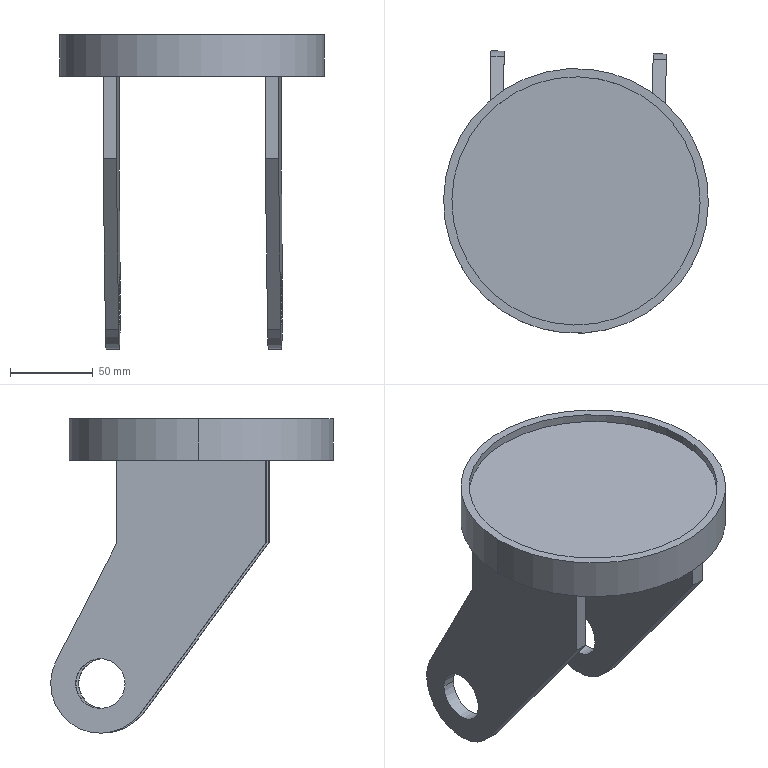Component | SolidWorks | FrontWheelAssembly-1_FrontWheelAccessory2-1 | 1 solid | 26 faces | box 160 x 170.95 x 190 mm | volume 607648 mm3 | plane 15 | cylinder 11 | commonest cylinder face diameters 30 x4 60 x3 150 x2 160 x2
build123d program:
from build123d import *

# Parameters (mm, degrees)
SKETCH1_R           = 80
SKETCH1_R_2         = 75
BOSS_EXTRUDE1_DEPTH = 5
BOSS_EXTRUDE2_START = 20
SKETCH2_R           = 80
BOSS_EXTRUDE2_DEPTH = 20
SKETCH3_R           = 15
BOSS_EXTRUDE3_DEPTH = 8


with BuildPart() as part:
    # Sketch1 → Boss-Extrude1 (new body)
    with BuildSketch(Plane(origin=(0, 0, 0), x_dir=(1, 0, 0), z_dir=(0, 1, 0))):
        with Locations(Location((0, 0, 0), (0, 0, 270))):
            Circle(SKETCH1_R)
        with Locations(Location((0, 0, 0), (0, 0, 270))):
            Circle(SKETCH1_R_2, mode=Mode.SUBTRACT)
    extrude(amount=BOSS_EXTRUDE1_DEPTH)

    # Sketch2 → Boss-Extrude2 (add)
    with BuildSketch(Plane.XZ.offset(BOSS_EXTRUDE2_START)):
        with Locations(Location((0, 0, 0), (0, 0, 270))):
            Circle(SKETCH2_R)
    extrude(amount=-BOSS_EXTRUDE2_DEPTH)

    # Sketch3 → Boss-Extrude3 (add)
    with BuildSketch(Plane.XY.offset(45)):
        with BuildLine():
            Line((50, -70), (50, -20))
            Line((50, -20), (-40.058, -20))
            Line((-40.058, -20), (-40.058, -70))
            Line((-40.058, -70), (35.866, -172.821))
            ThreePointArc((35.866, -172.821), (75.825, -180.487), (86.676, -141.273))
            Line((86.676, -141.273), (50, -70))
        make_face()
        with Locations((60, -155)):
            Circle(SKETCH3_R, mode=Mode.SUBTRACT)
    boss_extrude3 = extrude(amount=BOSS_EXTRUDE3_DEPTH)

    # Mirror1: Boss-Extrude3 across plane
    add(boss_extrude3.mirror(Plane.XY))


solid = part.part

# Placed as in the assembly
solid = solid.moved(Location((25.629, -64.9, 223), (90, 88.961, 0)))
STEP:
#1=COLOUR_RGB('',0.7922,0.8196,0.9333);
#2=FILL_AREA_STYLE_COLOUR('',#1);
#3=FILL_AREA_STYLE('',(#2));
#4=SURFACE_STYLE_FILL_AREA(#3);
#5=SURFACE_SIDE_STYLE('',(#4));
#6=SURFACE_STYLE_USAGE(.BOTH.,#5);
#7=PRESENTATION_STYLE_ASSIGNMENT((#6));
#8=CARTESIAN_POINT('',(-1.045,-0.7459,2.677));
#9=VERTEX_POINT('',#8);
#10=CARTESIAN_POINT('',(-1.024,0.435,2.677));
#11=VERTEX_POINT('',#10);
#12=CARTESIAN_POINT('',(-1.034,-0.1555,2.677));
#13=DIRECTION('',(0.9998,-0.01813,0.));
#14=DIRECTION('',(0.01813,0.9998,0.));
#15=AXIS2_PLACEMENT_3D('',#12,#13,#14);
#16=CIRCLE('',#15,0.5906);
#17=EDGE_CURVE('',#9,#11,#16,.T.);
#18=ORIENTED_EDGE('',*,*,#17,.F.);
#19=CARTESIAN_POINT('',(-0.7302,-0.7516,2.677));
#20=VERTEX_POINT('',#19);
#21=CARTESIAN_POINT('',(-1.045,-0.7459,2.677));
#22=DIRECTION('',(0.9998,-0.01813,0.));
#23=VECTOR('',#22,39.37);
#24=LINE('',#21,#23);
#25=EDGE_CURVE('',#9,#20,#24,.T.);
#26=ORIENTED_EDGE('',*,*,#25,.T.);
#27=CARTESIAN_POINT('',(-0.7088,0.4293,2.677));
#28=VERTEX_POINT('',#27);
#29=CARTESIAN_POINT('',(-0.7195,-0.1612,2.677));
#30=DIRECTION('',(0.9998,-0.01813,0.));
#31=DIRECTION('',(0.01813,0.9998,0.));
#32=AXIS2_PLACEMENT_3D('',#29,#30,#31);
#33=CIRCLE('',#32,0.5906);
#34=EDGE_CURVE('',#20,#28,#33,.T.);
#35=ORIENTED_EDGE('',*,*,#34,.T.);
#36=CARTESIAN_POINT('',(-1.024,0.435,2.677));
#37=DIRECTION('',(0.9998,-0.01813,0.));
#38=VECTOR('',#37,39.37);
#39=LINE('',#36,#38);
#40=EDGE_CURVE('',#11,#28,#39,.T.);
#41=ORIENTED_EDGE('',*,*,#40,.F.);
#42=EDGE_LOOP('',(#18,#26,#35,#41));
#43=FACE_OUTER_BOUND('',#42,.T.);
#44=CARTESIAN_POINT('',(-1.034,-0.1555,2.677));
#45=DIRECTION('',(0.9998,-0.01813,0.));
#46=DIRECTION('',(0.01813,0.9998,0.));
#47=AXIS2_PLACEMENT_3D('',#44,#45,#46);
#48=CYLINDRICAL_SURFACE('',#47,0.5906);
#49=ADVANCED_FACE('',(#43),#48,.F.);
#50=CARTESIAN_POINT('',(-1.052,-1.105,1.976));
#51=VERTEX_POINT('',#50);
#52=CARTESIAN_POINT('',(-1.013,1.025,2.677));
#53=VERTEX_POINT('',#52);
#54=CARTESIAN_POINT('',(-1.034,-0.1555,2.677));
#55=DIRECTION('',(0.9998,-0.01813,0.));
#56=DIRECTION('',(0.01813,0.9998,0.));
#57=AXIS2_PLACEMENT_3D('',#54,#55,#56);
#58=CIRCLE('',#57,1.181);
#59=EDGE_CURVE('',#51,#53,#58,.T.);
#60=ORIENTED_EDGE('',*,*,#59,.T.);
#61=CARTESIAN_POINT('',(-0.6981,1.02,2.677));
#62=VERTEX_POINT('',#61);
#63=CARTESIAN_POINT('',(-1.013,1.025,2.677));
#64=DIRECTION('',(0.9998,-0.01813,0.));
#65=VECTOR('',#64,39.37);
#66=LINE('',#63,#65);
#67=EDGE_CURVE('',#53,#62,#66,.T.);
#68=ORIENTED_EDGE('',*,*,#67,.T.);
#69=CARTESIAN_POINT('',(-0.7367,-1.111,1.976));
#70=VERTEX_POINT('',#69);
#71=CARTESIAN_POINT('',(-0.7195,-0.1612,2.677));
#72=DIRECTION('',(0.9998,-0.01813,0.));
#73=DIRECTION('',(0.01813,0.9998,0.));
#74=AXIS2_PLACEMENT_3D('',#71,#72,#73);
#75=CIRCLE('',#74,1.181);
#76=EDGE_CURVE('',#70,#62,#75,.T.);
#77=ORIENTED_EDGE('',*,*,#76,.F.);
#78=CARTESIAN_POINT('',(-1.052,-1.105,1.976));
#79=DIRECTION('',(0.9998,-0.01813,0.));
#80=VECTOR('',#79,39.37);
#81=LINE('',#78,#80);
#82=EDGE_CURVE('',#51,#70,#81,.T.);
#83=ORIENTED_EDGE('',*,*,#82,.F.);
#84=EDGE_LOOP('',(#60,#68,#77,#83));
#85=FACE_OUTER_BOUND('',#84,.T.);
#86=CARTESIAN_POINT('',(-1.034,-0.1555,2.677));
#87=DIRECTION('',(0.9998,-0.01813,0.));
#88=DIRECTION('',(0.01813,0.9998,0.));
#89=AXIS2_PLACEMENT_3D('',#86,#87,#88);
#90=CYLINDRICAL_SURFACE('',#89,1.181);
#91=ADVANCED_FACE('',(#85),#90,.T.);
#92=CARTESIAN_POINT('',(3.127,-0.8216,2.677));
#93=VERTEX_POINT('',#92);
#94=CARTESIAN_POINT('',(3.149,0.3593,2.677));
#95=VERTEX_POINT('',#94);
#96=CARTESIAN_POINT('',(3.138,-0.2311,2.677));
#97=DIRECTION('',(0.9998,-0.01813,0.));
#98=DIRECTION('',(0.01813,0.9998,0.));
#99=AXIS2_PLACEMENT_3D('',#96,#97,#98);
#100=CIRCLE('',#99,0.5906);
#101=EDGE_CURVE('',#93,#95,#100,.T.);
#102=ORIENTED_EDGE('',*,*,#101,.T.);
#103=CARTESIAN_POINT('',(2.834,0.365,2.677));
#104=VERTEX_POINT('',#103);
#105=CARTESIAN_POINT('',(3.149,0.3593,2.677));
#106=DIRECTION('',(-0.9998,0.01813,-0.));
#107=VECTOR('',#106,39.37);
#108=LINE('',#105,#107);
#109=EDGE_CURVE('',#95,#104,#108,.T.);
#110=ORIENTED_EDGE('',*,*,#109,.T.);
#111=CARTESIAN_POINT('',(2.813,-0.8159,2.677));
#112=VERTEX_POINT('',#111);
#113=CARTESIAN_POINT('',(2.823,-0.2254,2.677));
#114=DIRECTION('',(0.9998,-0.01813,0.));
#115=DIRECTION('',(0.01813,0.9998,0.));
#116=AXIS2_PLACEMENT_3D('',#113,#114,#115);
#117=CIRCLE('',#116,0.5906);
#118=EDGE_CURVE('',#112,#104,#117,.T.);
#119=ORIENTED_EDGE('',*,*,#118,.F.);
#120=CARTESIAN_POINT('',(3.127,-0.8216,2.677));
#121=DIRECTION('',(-0.9998,0.01813,-0.));
#122=VECTOR('',#121,39.37);
#123=LINE('',#120,#122);
#124=EDGE_CURVE('',#93,#112,#123,.T.);
#125=ORIENTED_EDGE('',*,*,#124,.F.);
#126=EDGE_LOOP('',(#102,#110,#119,#125));
#127=FACE_OUTER_BOUND('',#126,.T.);
#128=CARTESIAN_POINT('',(3.138,-0.2311,2.677));
#129=DIRECTION('',(-0.9998,0.01813,-0.));
#130=DIRECTION('',(-0.01813,-0.9998,-0.));
#131=AXIS2_PLACEMENT_3D('',#128,#129,#130);
#132=CYLINDRICAL_SURFACE('',#131,0.5906);
#133=ADVANCED_FACE('',(#127),#132,.F.);
#134=CARTESIAN_POINT('',(-1.943,-2.502,8.976));
#135=VERTEX_POINT('',#134);
#136=CARTESIAN_POINT('',(3.961,-2.609,8.976));
#137=VERTEX_POINT('',#136);
#138=CARTESIAN_POINT('',(1.009,-2.555,8.976));
#139=DIRECTION('',(-0.,-0.,1.));
#140=DIRECTION('',(0.9998,-0.01813,0.));
#141=AXIS2_PLACEMENT_3D('',#138,#139,#140);
#142=CIRCLE('',#141,2.953);
#143=EDGE_CURVE('',#135,#137,#142,.T.);
#144=ORIENTED_EDGE('',*,*,#143,.T.);
#145=CARTESIAN_POINT('',(3.961,-2.609,8.78));
#146=VERTEX_POINT('',#145);
#147=CARTESIAN_POINT('',(3.961,-2.609,8.976));
#148=DIRECTION('',(0.,0.,-1.));
#149=VECTOR('',#148,39.37);
#150=LINE('',#147,#149);
#151=EDGE_CURVE('',#137,#146,#150,.T.);
#152=ORIENTED_EDGE('',*,*,#151,.T.);
#153=CARTESIAN_POINT('',(-1.943,-2.502,8.78));
#154=VERTEX_POINT('',#153);
#155=CARTESIAN_POINT('',(1.009,-2.555,8.78));
#156=DIRECTION('',(-0.,-0.,1.));
#157=DIRECTION('',(0.9998,-0.01813,0.));
#158=AXIS2_PLACEMENT_3D('',#155,#156,#157);
#159=CIRCLE('',#158,2.953);
#160=EDGE_CURVE('',#154,#146,#159,.T.);
#161=ORIENTED_EDGE('',*,*,#160,.F.);
#162=CARTESIAN_POINT('',(-1.943,-2.502,8.976));
#163=DIRECTION('',(0.,0.,-1.));
#164=VECTOR('',#163,39.37);
#165=LINE('',#162,#164);
#166=EDGE_CURVE('',#135,#154,#165,.T.);
#167=ORIENTED_EDGE('',*,*,#166,.F.);
#168=EDGE_LOOP('',(#144,#152,#161,#167));
#169=FACE_OUTER_BOUND('',#168,.T.);
#170=CARTESIAN_POINT('',(1.009,-2.555,8.976));
#171=DIRECTION('',(0.,0.,-1.));
#172=DIRECTION('',(-0.9998,0.01813,-0.));
#173=AXIS2_PLACEMENT_3D('',#170,#171,#172);
#174=CYLINDRICAL_SURFACE('',#173,2.953);
#175=ADVANCED_FACE('',(#169),#174,.F.);
#176=CARTESIAN_POINT('',(4.158,-2.612,8.976));
#177=VERTEX_POINT('',#176);
#178=CARTESIAN_POINT('',(-2.14,-2.498,8.976));
#179=VERTEX_POINT('',#178);
#180=CARTESIAN_POINT('',(1.009,-2.555,8.976));
#181=DIRECTION('',(-0.,-0.,1.));
#182=DIRECTION('',(0.9998,-0.01813,0.));
#183=AXIS2_PLACEMENT_3D('',#180,#181,#182);
#184=CIRCLE('',#183,3.15);
#185=EDGE_CURVE('',#177,#179,#184,.T.);
#186=ORIENTED_EDGE('',*,*,#185,.F.);
#187=CARTESIAN_POINT('',(4.158,-2.612,7.992));
#188=VERTEX_POINT('',#187);
#189=CARTESIAN_POINT('',(4.158,-2.612,8.976));
#190=DIRECTION('',(0.,0.,-1.));
#191=VECTOR('',#190,39.37);
#192=LINE('',#189,#191);
#193=EDGE_CURVE('',#177,#188,#192,.T.);
#194=ORIENTED_EDGE('',*,*,#193,.T.);
#195=CARTESIAN_POINT('',(-2.14,-2.498,7.992));
#196=VERTEX_POINT('',#195);
#197=CARTESIAN_POINT('',(1.009,-2.555,7.992));
#198=DIRECTION('',(0.,0.,-1.));
#199=DIRECTION('',(-0.9998,0.01813,-0.));
#200=AXIS2_PLACEMENT_3D('',#197,#198,#199);
#201=CIRCLE('',#200,3.15);
#202=EDGE_CURVE('',#196,#188,#201,.T.);
#203=ORIENTED_EDGE('',*,*,#202,.F.);
#204=CARTESIAN_POINT('',(-2.14,-2.498,8.976));
#205=DIRECTION('',(0.,0.,-1.));
#206=VECTOR('',#205,39.37);
#207=LINE('',#204,#206);
#208=EDGE_CURVE('',#179,#196,#207,.T.);
#209=ORIENTED_EDGE('',*,*,#208,.F.);
#210=EDGE_LOOP('',(#186,#194,#203,#209));
#211=FACE_OUTER_BOUND('',#210,.T.);
#212=CARTESIAN_POINT('',(1.009,-2.555,8.976));
#213=DIRECTION('',(0.,0.,-1.));
#214=DIRECTION('',(-0.9998,0.01813,-0.));
#215=AXIS2_PLACEMENT_3D('',#212,#213,#214);
#216=CYLINDRICAL_SURFACE('',#215,3.15);
#217=ADVANCED_FACE('',(#211),#216,.T.);
#218=CARTESIAN_POINT('',(1.009,-2.555,8.976));
#219=DIRECTION('',(-0.,-0.,1.));
#220=DIRECTION('',(0.9998,-0.01813,0.));
#221=AXIS2_PLACEMENT_3D('',#218,#219,#220);
#222=CIRCLE('',#221,3.15);
#223=EDGE_CURVE('',#179,#177,#222,.T.);
#224=ORIENTED_EDGE('',*,*,#223,.T.);
#225=ORIENTED_EDGE('',*,*,#185,.T.);
#226=EDGE_LOOP('',(#224,#225));
#227=FACE_OUTER_BOUND('',#226,.T.);
#228=ORIENTED_EDGE('',*,*,#143,.F.);
#229=CARTESIAN_POINT('',(1.009,-2.555,8.976));
#230=DIRECTION('',(-0.,-0.,1.));
#231=DIRECTION('',(0.9998,-0.01813,0.));
#232=AXIS2_PLACEMENT_3D('',#229,#230,#231);
#233=CIRCLE('',#232,2.953);
#234=EDGE_CURVE('',#137,#135,#233,.T.);
#235=ORIENTED_EDGE('',*,*,#234,.F.);
#236=EDGE_LOOP('',(#228,#235));
#237=FACE_BOUND('',#236,.T.);
#238=CARTESIAN_POINT('',(1.009,-2.555,8.976));
#239=DIRECTION('',(-0.,-0.,1.));
#240=DIRECTION('',(0.9998,-0.01813,0.));
#241=AXIS2_PLACEMENT_3D('',#238,#239,#240);
#242=PLANE('',#241);
#243=ADVANCED_FACE('',(#227,#237),#242,.T.);
#244=ORIENTED_EDGE('',*,*,#193,.F.);
#245=ORIENTED_EDGE('',*,*,#223,.F.);
#246=ORIENTED_EDGE('',*,*,#208,.T.);
#247=CARTESIAN_POINT('',(1.009,-2.555,7.992));
#248=DIRECTION('',(0.,0.,-1.));
#249=DIRECTION('',(-0.9998,0.01813,-0.));
#250=AXIS2_PLACEMENT_3D('',#247,#248,#249);
#251=CIRCLE('',#250,3.15);
#252=EDGE_CURVE('',#188,#196,#251,.T.);
#253=ORIENTED_EDGE('',*,*,#252,.F.);
#254=EDGE_LOOP('',(#244,#245,#246,#253));
#255=FACE_OUTER_BOUND('',#254,.T.);
#256=CARTESIAN_POINT('',(1.009,-2.555,8.976));
#257=DIRECTION('',(0.,0.,-1.));
#258=DIRECTION('',(-0.9998,0.01813,-0.));
#259=AXIS2_PLACEMENT_3D('',#256,#257,#258);
#260=CYLINDRICAL_SURFACE('',#259,3.15);
#261=ADVANCED_FACE('',(#255),#260,.T.);
#262=ORIENTED_EDGE('',*,*,#151,.F.);
#263=ORIENTED_EDGE('',*,*,#234,.T.);
#264=ORIENTED_EDGE('',*,*,#166,.T.);
#265=CARTESIAN_POINT('',(1.009,-2.555,8.78));
#266=DIRECTION('',(-0.,-0.,1.));
#267=DIRECTION('',(0.9998,-0.01813,0.));
#268=AXIS2_PLACEMENT_3D('',#265,#266,#267);
#269=CIRCLE('',#268,2.953);
#270=EDGE_CURVE('',#146,#154,#269,.T.);
#271=ORIENTED_EDGE('',*,*,#270,.F.);
#272=EDGE_LOOP('',(#262,#263,#264,#271));
#273=FACE_OUTER_BOUND('',#272,.T.);
#274=CARTESIAN_POINT('',(1.009,-2.555,8.976));
#275=DIRECTION('',(0.,0.,-1.));
#276=DIRECTION('',(-0.9998,0.01813,-0.));
#277=AXIS2_PLACEMENT_3D('',#274,#275,#276);
#278=CYLINDRICAL_SURFACE('',#277,2.953);
#279=ADVANCED_FACE('',(#273),#278,.F.);
#280=ORIENTED_EDGE('',*,*,#160,.T.);
#281=ORIENTED_EDGE('',*,*,#270,.T.);
#282=EDGE_LOOP('',(#280,#281));
#283=FACE_OUTER_BOUND('',#282,.T.);
#284=CARTESIAN_POINT('',(1.009,-2.555,8.78));
#285=DIRECTION('',(0.,0.,-1.));
#286=DIRECTION('',(-0.9998,0.01813,-0.));
#287=AXIS2_PLACEMENT_3D('',#284,#285,#286);
#288=PLANE('',#287);
#289=ADVANCED_FACE('',(#283),#288,.F.);
#290=CARTESIAN_POINT('',(-1.106,-4.094,7.992));
#291=VERTEX_POINT('',#290);
#292=CARTESIAN_POINT('',(-1.042,-0.5491,7.992));
#293=VERTEX_POINT('',#292);
#294=CARTESIAN_POINT('',(-1.077,-2.517,7.992));
#295=DIRECTION('',(0.01813,0.9998,0.));
#296=VECTOR('',#295,39.37);
#297=LINE('',#294,#296);
#298=EDGE_CURVE('',#291,#293,#297,.T.);
#299=ORIENTED_EDGE('',*,*,#298,.F.);
#300=CARTESIAN_POINT('',(-0.7909,-4.1,7.992));
#301=VERTEX_POINT('',#300);
#302=CARTESIAN_POINT('',(-1.106,-4.094,7.992));
#303=DIRECTION('',(0.9998,-0.01813,0.));
#304=VECTOR('',#303,39.37);
#305=LINE('',#302,#304);
#306=EDGE_CURVE('',#291,#301,#305,.T.);
#307=ORIENTED_EDGE('',*,*,#306,.T.);
#308=CARTESIAN_POINT('',(-0.7266,-0.5548,7.992));
#309=VERTEX_POINT('',#308);
#310=CARTESIAN_POINT('',(-0.7623,-2.523,7.992));
#311=DIRECTION('',(0.01813,0.9998,0.));
#312=VECTOR('',#311,39.37);
#313=LINE('',#310,#312);
#314=EDGE_CURVE('',#301,#309,#313,.T.);
#315=ORIENTED_EDGE('',*,*,#314,.T.);
#316=CARTESIAN_POINT('',(-1.042,-0.5491,7.992));
#317=DIRECTION('',(0.9998,-0.01813,0.));
#318=VECTOR('',#317,39.37);
#319=LINE('',#316,#318);
#320=EDGE_CURVE('',#293,#309,#319,.T.);
#321=ORIENTED_EDGE('',*,*,#320,.F.);
#322=EDGE_LOOP('',(#299,#307,#315,#321));
#323=FACE_BOUND('',#322,.T.);
#324=CARTESIAN_POINT('',(3.067,-4.17,7.992));
#325=VERTEX_POINT('',#324);
#326=CARTESIAN_POINT('',(3.131,-0.6248,7.992));
#327=VERTEX_POINT('',#326);
#328=CARTESIAN_POINT('',(3.095,-2.593,7.992));
#329=DIRECTION('',(0.01813,0.9998,0.));
#330=VECTOR('',#329,39.37);
#331=LINE('',#328,#330);
#332=EDGE_CURVE('',#325,#327,#331,.T.);
#333=ORIENTED_EDGE('',*,*,#332,.T.);
#334=CARTESIAN_POINT('',(2.816,-0.6191,7.992));
#335=VERTEX_POINT('',#334);
#336=CARTESIAN_POINT('',(3.131,-0.6248,7.992));
#337=DIRECTION('',(-0.9998,0.01813,-0.));
#338=VECTOR('',#337,39.37);
#339=LINE('',#336,#338);
#340=EDGE_CURVE('',#327,#335,#339,.T.);
#341=ORIENTED_EDGE('',*,*,#340,.T.);
#342=CARTESIAN_POINT('',(2.752,-4.164,7.992));
#343=VERTEX_POINT('',#342);
#344=CARTESIAN_POINT('',(2.78,-2.587,7.992));
#345=DIRECTION('',(0.01813,0.9998,0.));
#346=VECTOR('',#345,39.37);
#347=LINE('',#344,#346);
#348=EDGE_CURVE('',#343,#335,#347,.T.);
#349=ORIENTED_EDGE('',*,*,#348,.F.);
#350=CARTESIAN_POINT('',(3.067,-4.17,7.992));
#351=DIRECTION('',(-0.9998,0.01813,-0.));
#352=VECTOR('',#351,39.37);
#353=LINE('',#350,#352);
#354=EDGE_CURVE('',#325,#343,#353,.T.);
#355=ORIENTED_EDGE('',*,*,#354,.F.);
#356=EDGE_LOOP('',(#333,#341,#349,#355));
#357=FACE_BOUND('',#356,.T.);
#358=ORIENTED_EDGE('',*,*,#202,.T.);
#359=ORIENTED_EDGE('',*,*,#252,.T.);
#360=EDGE_LOOP('',(#358,#359));
#361=FACE_OUTER_BOUND('',#360,.T.);
#362=CARTESIAN_POINT('',(1.009,-2.555,7.992));
#363=DIRECTION('',(0.,0.,-1.));
#364=DIRECTION('',(-0.9998,0.01813,-0.));
#365=AXIS2_PLACEMENT_3D('',#362,#363,#364);
#366=PLANE('',#365);
#367=ADVANCED_FACE('',(#323,#357,#361),#366,.T.);
#368=CARTESIAN_POINT('',(2.752,-4.164,6.024));
#369=VERTEX_POINT('',#368);
#370=CARTESIAN_POINT('',(2.806,-1.175,1.976));
#371=VERTEX_POINT('',#370);
#372=CARTESIAN_POINT('',(2.738,-4.924,7.053));
#373=DIRECTION('',(0.01077,0.5939,-0.8045));
#374=VECTOR('',#373,39.37);
#375=LINE('',#372,#374);
#376=EDGE_CURVE('',#369,#371,#375,.T.);
#377=ORIENTED_EDGE('',*,*,#376,.T.);
#378=CARTESIAN_POINT('',(3.121,-1.181,1.976));
#379=VERTEX_POINT('',#378);
#380=CARTESIAN_POINT('',(3.121,-1.181,1.976));
#381=DIRECTION('',(-0.9998,0.01813,-0.));
#382=VECTOR('',#381,39.37);
#383=LINE('',#380,#382);
#384=EDGE_CURVE('',#379,#371,#383,.T.);
#385=ORIENTED_EDGE('',*,*,#384,.F.);
#386=CARTESIAN_POINT('',(3.067,-4.17,6.024));
#387=VERTEX_POINT('',#386);
#388=CARTESIAN_POINT('',(3.053,-4.93,7.053));
#389=DIRECTION('',(0.01077,0.5939,-0.8045));
#390=VECTOR('',#389,39.37);
#391=LINE('',#388,#390);
#392=EDGE_CURVE('',#387,#379,#391,.T.);
#393=ORIENTED_EDGE('',*,*,#392,.F.);
#394=CARTESIAN_POINT('',(3.067,-4.17,6.024));
#395=DIRECTION('',(-0.9998,0.01813,-0.));
#396=VECTOR('',#395,39.37);
#397=LINE('',#394,#396);
#398=EDGE_CURVE('',#387,#369,#397,.T.);
#399=ORIENTED_EDGE('',*,*,#398,.T.);
#400=EDGE_LOOP('',(#377,#385,#393,#399));
#401=FACE_OUTER_BOUND('',#400,.T.);
#402=CARTESIAN_POINT('',(3.053,-4.93,7.053));
#403=DIRECTION('',(0.01459,0.8043,0.594));
#404=DIRECTION('',(-0.01077,-0.5939,0.8045));
#405=AXIS2_PLACEMENT_3D('',#402,#403,#404);
#406=PLANE('',#405);
#407=ADVANCED_FACE('',(#401),#406,.F.);
#408=CARTESIAN_POINT('',(2.842,0.8246,3.218));
#409=VERTEX_POINT('',#408);
#410=CARTESIAN_POINT('',(2.823,-0.2254,2.677));
#411=DIRECTION('',(0.9998,-0.01813,0.));
#412=DIRECTION('',(0.01813,0.9998,0.));
#413=AXIS2_PLACEMENT_3D('',#410,#411,#412);
#414=CIRCLE('',#413,1.181);
#415=EDGE_CURVE('',#371,#409,#414,.T.);
#416=ORIENTED_EDGE('',*,*,#415,.T.);
#417=CARTESIAN_POINT('',(3.157,0.8189,3.218));
#418=VERTEX_POINT('',#417);
#419=CARTESIAN_POINT('',(3.157,0.8189,3.218));
#420=DIRECTION('',(-0.9998,0.01813,-0.));
#421=VECTOR('',#420,39.37);
#422=LINE('',#419,#421);
#423=EDGE_CURVE('',#418,#409,#422,.T.);
#424=ORIENTED_EDGE('',*,*,#423,.F.);
#425=CARTESIAN_POINT('',(3.138,-0.2311,2.677));
#426=DIRECTION('',(0.9998,-0.01813,0.));
#427=DIRECTION('',(0.01813,0.9998,0.));
#428=AXIS2_PLACEMENT_3D('',#425,#426,#427);
#429=CIRCLE('',#428,1.181);
#430=EDGE_CURVE('',#379,#418,#429,.T.);
#431=ORIENTED_EDGE('',*,*,#430,.F.);
#432=ORIENTED_EDGE('',*,*,#384,.T.);
#433=EDGE_LOOP('',(#416,#424,#431,#432));
#434=FACE_OUTER_BOUND('',#433,.T.);
#435=CARTESIAN_POINT('',(3.138,-0.2311,2.677));
#436=DIRECTION('',(-0.9998,0.01813,-0.));
#437=DIRECTION('',(-0.01813,-0.9998,-0.));
#438=AXIS2_PLACEMENT_3D('',#435,#436,#437);
#439=CYLINDRICAL_SURFACE('',#438,1.181);
#440=ADVANCED_FACE('',(#434),#439,.T.);
#441=CARTESIAN_POINT('',(2.816,-0.6191,6.024));
#442=VERTEX_POINT('',#441);
#443=CARTESIAN_POINT('',(2.788,-2.152,9.003));
#444=DIRECTION('',(0.008298,0.4575,-0.8892));
#445=VECTOR('',#444,39.37);
#446=LINE('',#443,#445);
#447=EDGE_CURVE('',#442,#409,#446,.T.);
#448=ORIENTED_EDGE('',*,*,#447,.F.);
#449=CARTESIAN_POINT('',(3.131,-0.6248,6.024));
#450=VERTEX_POINT('',#449);
#451=CARTESIAN_POINT('',(3.131,-0.6248,6.024));
#452=DIRECTION('',(-0.9998,0.01813,-0.));
#453=VECTOR('',#452,39.37);
#454=LINE('',#451,#453);
#455=EDGE_CURVE('',#450,#442,#454,.T.);
#456=ORIENTED_EDGE('',*,*,#455,.F.);
#457=CARTESIAN_POINT('',(3.103,-2.158,9.003));
#458=DIRECTION('',(0.008298,0.4575,-0.8892));
#459=VECTOR('',#458,39.37);
#460=LINE('',#457,#459);
#461=EDGE_CURVE('',#450,#418,#460,.T.);
#462=ORIENTED_EDGE('',*,*,#461,.T.);
#463=ORIENTED_EDGE('',*,*,#423,.T.);
#464=EDGE_LOOP('',(#448,#456,#462,#463));
#465=FACE_OUTER_BOUND('',#464,.T.);
#466=CARTESIAN_POINT('',(3.103,-2.158,9.003));
#467=DIRECTION('',(0.01613,0.889,0.4576));
#468=DIRECTION('',(-0.008298,-0.4575,0.8892));
#469=AXIS2_PLACEMENT_3D('',#466,#467,#468);
#470=PLANE('',#469);
#471=ADVANCED_FACE('',(#465),#470,.T.);
#472=CARTESIAN_POINT('',(2.816,-0.6191,8.78));
#473=DIRECTION('',(0.,0.,-1.));
#474=VECTOR('',#473,39.37);
#475=LINE('',#472,#474);
#476=EDGE_CURVE('',#335,#442,#475,.T.);
#477=ORIENTED_EDGE('',*,*,#476,.F.);
#478=ORIENTED_EDGE('',*,*,#340,.F.);
#479=CARTESIAN_POINT('',(3.131,-0.6248,8.78));
#480=DIRECTION('',(0.,0.,-1.));
#481=VECTOR('',#480,39.37);
#482=LINE('',#479,#481);
#483=EDGE_CURVE('',#327,#450,#482,.T.);
#484=ORIENTED_EDGE('',*,*,#483,.T.);
#485=ORIENTED_EDGE('',*,*,#455,.T.);
#486=EDGE_LOOP('',(#477,#478,#484,#485));
#487=FACE_OUTER_BOUND('',#486,.T.);
#488=CARTESIAN_POINT('',(3.131,-0.6248,8.78));
#489=DIRECTION('',(0.01813,0.9998,0.));
#490=DIRECTION('',(-0.,-0.,1.));
#491=AXIS2_PLACEMENT_3D('',#488,#489,#490);
#492=PLANE('',#491);
#493=ADVANCED_FACE('',(#487),#492,.T.);
#494=CARTESIAN_POINT('',(2.752,-4.164,8.78));
#495=DIRECTION('',(0.,0.,-1.));
#496=VECTOR('',#495,39.37);
#497=LINE('',#494,#496);
#498=EDGE_CURVE('',#343,#369,#497,.T.);
#499=ORIENTED_EDGE('',*,*,#498,.T.);
#500=ORIENTED_EDGE('',*,*,#398,.F.);
#501=CARTESIAN_POINT('',(3.067,-4.17,8.78));
#502=DIRECTION('',(0.,0.,-1.));
#503=VECTOR('',#502,39.37);
#504=LINE('',#501,#503);
#505=EDGE_CURVE('',#325,#387,#504,.T.);
#506=ORIENTED_EDGE('',*,*,#505,.F.);
#507=ORIENTED_EDGE('',*,*,#354,.T.);
#508=EDGE_LOOP('',(#499,#500,#506,#507));
#509=FACE_OUTER_BOUND('',#508,.T.);
#510=CARTESIAN_POINT('',(3.067,-4.17,8.78));
#511=DIRECTION('',(0.01813,0.9998,0.));
#512=DIRECTION('',(-0.,-0.,1.));
#513=AXIS2_PLACEMENT_3D('',#510,#511,#512);
#514=PLANE('',#513);
#515=ADVANCED_FACE('',(#509),#514,.F.);
#516=ORIENTED_EDGE('',*,*,#109,.F.);
#517=CARTESIAN_POINT('',(3.138,-0.2311,2.677));
#518=DIRECTION('',(0.9998,-0.01813,0.));
#519=DIRECTION('',(0.01813,0.9998,0.));
#520=AXIS2_PLACEMENT_3D('',#517,#518,#519);
#521=CIRCLE('',#520,0.5906);
#522=EDGE_CURVE('',#95,#93,#521,.T.);
#523=ORIENTED_EDGE('',*,*,#522,.T.);
#524=ORIENTED_EDGE('',*,*,#124,.T.);
#525=CARTESIAN_POINT('',(2.823,-0.2254,2.677));
#526=DIRECTION('',(0.9998,-0.01813,0.));
#527=DIRECTION('',(0.01813,0.9998,0.));
#528=AXIS2_PLACEMENT_3D('',#525,#526,#527);
#529=CIRCLE('',#528,0.5906);
#530=EDGE_CURVE('',#104,#112,#529,.T.);
#531=ORIENTED_EDGE('',*,*,#530,.F.);
#532=EDGE_LOOP('',(#516,#523,#524,#531));
#533=FACE_OUTER_BOUND('',#532,.T.);
#534=CARTESIAN_POINT('',(3.138,-0.2311,2.677));
#535=DIRECTION('',(-0.9998,0.01813,-0.));
#536=DIRECTION('',(-0.01813,-0.9998,-0.));
#537=AXIS2_PLACEMENT_3D('',#534,#535,#536);
#538=CYLINDRICAL_SURFACE('',#537,0.5906);
#539=ADVANCED_FACE('',(#533),#538,.F.);
#540=ORIENTED_EDGE('',*,*,#392,.T.);
#541=ORIENTED_EDGE('',*,*,#430,.T.);
#542=ORIENTED_EDGE('',*,*,#461,.F.);
#543=ORIENTED_EDGE('',*,*,#483,.F.);
#544=ORIENTED_EDGE('',*,*,#332,.F.);
#545=ORIENTED_EDGE('',*,*,#505,.T.);
#546=EDGE_LOOP('',(#540,#541,#542,#543,#544,#545));
#547=FACE_OUTER_BOUND('',#546,.T.);
#548=ORIENTED_EDGE('',*,*,#101,.F.);
#549=ORIENTED_EDGE('',*,*,#522,.F.);
#550=EDGE_LOOP('',(#548,#549));
#551=FACE_BOUND('',#550,.T.);
#552=CARTESIAN_POINT('',(3.095,-2.593,8.78));
#553=DIRECTION('',(0.9998,-0.01813,0.));
#554=DIRECTION('',(0.01813,0.9998,0.));
#555=AXIS2_PLACEMENT_3D('',#552,#553,#554);
#556=PLANE('',#555);
#557=ADVANCED_FACE('',(#547,#551),#556,.T.);
#558=ORIENTED_EDGE('',*,*,#376,.F.);
#559=ORIENTED_EDGE('',*,*,#498,.F.);
#560=ORIENTED_EDGE('',*,*,#348,.T.);
#561=ORIENTED_EDGE('',*,*,#476,.T.);
#562=ORIENTED_EDGE('',*,*,#447,.T.);
#563=ORIENTED_EDGE('',*,*,#415,.F.);
#564=EDGE_LOOP('',(#558,#559,#560,#561,#562,#563));
#565=FACE_OUTER_BOUND('',#564,.T.);
#566=ORIENTED_EDGE('',*,*,#118,.T.);
#567=ORIENTED_EDGE('',*,*,#530,.T.);
#568=EDGE_LOOP('',(#566,#567));
#569=FACE_BOUND('',#568,.T.);
#570=CARTESIAN_POINT('',(2.78,-2.587,8.78));
#571=DIRECTION('',(0.9998,-0.01813,0.));
#572=DIRECTION('',(0.01813,0.9998,0.));
#573=AXIS2_PLACEMENT_3D('',#570,#571,#572);
#574=PLANE('',#573);
#575=ADVANCED_FACE('',(#565,#569),#574,.F.);
#576=CARTESIAN_POINT('',(-0.7909,-4.1,6.024));
#577=VERTEX_POINT('',#576);
#578=CARTESIAN_POINT('',(-0.8047,-4.86,7.053));
#579=DIRECTION('',(0.01077,0.5939,-0.8045));
#580=VECTOR('',#579,39.37);
#581=LINE('',#578,#580);
#582=EDGE_CURVE('',#577,#70,#581,.T.);
#583=ORIENTED_EDGE('',*,*,#582,.F.);
#584=CARTESIAN_POINT('',(-1.106,-4.094,6.024));
#585=VERTEX_POINT('',#584);
#586=CARTESIAN_POINT('',(-1.106,-4.094,6.024));
#587=DIRECTION('',(0.9998,-0.01813,0.));
#588=VECTOR('',#587,39.37);
#589=LINE('',#586,#588);
#590=EDGE_CURVE('',#585,#577,#589,.T.);
#591=ORIENTED_EDGE('',*,*,#590,.F.);
#592=CARTESIAN_POINT('',(-1.12,-4.854,7.053));
#593=DIRECTION('',(0.01077,0.5939,-0.8045));
#594=VECTOR('',#593,39.37);
#595=LINE('',#592,#594);
#596=EDGE_CURVE('',#585,#51,#595,.T.);
#597=ORIENTED_EDGE('',*,*,#596,.T.);
#598=ORIENTED_EDGE('',*,*,#82,.T.);
#599=EDGE_LOOP('',(#583,#591,#597,#598));
#600=FACE_OUTER_BOUND('',#599,.T.);
#601=CARTESIAN_POINT('',(-1.12,-4.854,7.053));
#602=DIRECTION('',(-0.01459,-0.8043,-0.594));
#603=DIRECTION('',(0.01077,0.5939,-0.8045));
#604=AXIS2_PLACEMENT_3D('',#601,#602,#603);
#605=PLANE('',#604);
#606=ADVANCED_FACE('',(#600),#605,.T.);
#607=CARTESIAN_POINT('',(-0.7909,-4.1,8.78));
#608=DIRECTION('',(0.,0.,-1.));
#609=VECTOR('',#608,39.37);
#610=LINE('',#607,#609);
#611=EDGE_CURVE('',#301,#577,#610,.T.);
#612=ORIENTED_EDGE('',*,*,#611,.F.);
#613=ORIENTED_EDGE('',*,*,#306,.F.);
#614=CARTESIAN_POINT('',(-1.106,-4.094,8.78));
#615=DIRECTION('',(0.,0.,-1.));
#616=VECTOR('',#615,39.37);
#617=LINE('',#614,#616);
#618=EDGE_CURVE('',#291,#585,#617,.T.);
#619=ORIENTED_EDGE('',*,*,#618,.T.);
#620=ORIENTED_EDGE('',*,*,#590,.T.);
#621=EDGE_LOOP('',(#612,#613,#619,#620));
#622=FACE_OUTER_BOUND('',#621,.T.);
#623=CARTESIAN_POINT('',(-1.106,-4.094,8.78));
#624=DIRECTION('',(-0.01813,-0.9998,-0.));
#625=DIRECTION('',(0.,0.,-1.));
#626=AXIS2_PLACEMENT_3D('',#623,#624,#625);
#627=PLANE('',#626);
#628=ADVANCED_FACE('',(#622),#627,.T.);
#629=CARTESIAN_POINT('',(-0.7266,-0.5548,6.024));
#630=VERTEX_POINT('',#629);
#631=CARTESIAN_POINT('',(-0.7266,-0.5548,8.78));
#632=DIRECTION('',(0.,0.,-1.));
#633=VECTOR('',#632,39.37);
#634=LINE('',#631,#633);
#635=EDGE_CURVE('',#309,#630,#634,.T.);
#636=ORIENTED_EDGE('',*,*,#635,.T.);
#637=CARTESIAN_POINT('',(-1.042,-0.5491,6.024));
#638=VERTEX_POINT('',#637);
#639=CARTESIAN_POINT('',(-1.042,-0.5491,6.024));
#640=DIRECTION('',(0.9998,-0.01813,0.));
#641=VECTOR('',#640,39.37);
#642=LINE('',#639,#641);
#643=EDGE_CURVE('',#638,#630,#642,.T.);
#644=ORIENTED_EDGE('',*,*,#643,.F.);
#645=CARTESIAN_POINT('',(-1.042,-0.5491,8.78));
#646=DIRECTION('',(0.,0.,-1.));
#647=VECTOR('',#646,39.37);
#648=LINE('',#645,#647);
#649=EDGE_CURVE('',#293,#638,#648,.T.);
#650=ORIENTED_EDGE('',*,*,#649,.F.);
#651=ORIENTED_EDGE('',*,*,#320,.T.);
#652=EDGE_LOOP('',(#636,#644,#650,#651));
#653=FACE_OUTER_BOUND('',#652,.T.);
#654=CARTESIAN_POINT('',(-1.042,-0.5491,8.78));
#655=DIRECTION('',(-0.01813,-0.9998,-0.));
#656=DIRECTION('',(0.,0.,-1.));
#657=AXIS2_PLACEMENT_3D('',#654,#655,#656);
#658=PLANE('',#657);
#659=ADVANCED_FACE('',(#653),#658,.F.);
#660=CARTESIAN_POINT('',(-0.7005,0.8889,3.218));
#661=VERTEX_POINT('',#660);
#662=CARTESIAN_POINT('',(-0.7544,-2.088,9.003));
#663=DIRECTION('',(0.008298,0.4575,-0.8892));
#664=VECTOR('',#663,39.37);
#665=LINE('',#662,#664);
#666=EDGE_CURVE('',#630,#661,#665,.T.);
#667=ORIENTED_EDGE('',*,*,#666,.T.);
#668=CARTESIAN_POINT('',(-1.015,0.8946,3.218));
#669=VERTEX_POINT('',#668);
#670=CARTESIAN_POINT('',(-1.015,0.8946,3.218));
#671=DIRECTION('',(0.9998,-0.01813,0.));
#672=VECTOR('',#671,39.37);
#673=LINE('',#670,#672);
#674=EDGE_CURVE('',#669,#661,#673,.T.);
#675=ORIENTED_EDGE('',*,*,#674,.F.);
#676=CARTESIAN_POINT('',(-1.069,-2.082,9.003));
#677=DIRECTION('',(0.008298,0.4575,-0.8892));
#678=VECTOR('',#677,39.37);
#679=LINE('',#676,#678);
#680=EDGE_CURVE('',#638,#669,#679,.T.);
#681=ORIENTED_EDGE('',*,*,#680,.F.);
#682=ORIENTED_EDGE('',*,*,#643,.T.);
#683=EDGE_LOOP('',(#667,#675,#681,#682));
#684=FACE_OUTER_BOUND('',#683,.T.);
#685=CARTESIAN_POINT('',(-1.069,-2.082,9.003));
#686=DIRECTION('',(-0.01613,-0.889,-0.4576));
#687=DIRECTION('',(0.008298,0.4575,-0.8892));
#688=AXIS2_PLACEMENT_3D('',#685,#686,#687);
#689=PLANE('',#688);
#690=ADVANCED_FACE('',(#684),#689,.F.);
#691=ORIENTED_EDGE('',*,*,#67,.F.);
#692=CARTESIAN_POINT('',(-1.034,-0.1555,2.677));
#693=DIRECTION('',(0.9998,-0.01813,0.));
#694=DIRECTION('',(0.01813,0.9998,0.));
#695=AXIS2_PLACEMENT_3D('',#692,#693,#694);
#696=CIRCLE('',#695,1.181);
#697=EDGE_CURVE('',#53,#669,#696,.T.);
#698=ORIENTED_EDGE('',*,*,#697,.T.);
#699=ORIENTED_EDGE('',*,*,#674,.T.);
#700=CARTESIAN_POINT('',(-0.7195,-0.1612,2.677));
#701=DIRECTION('',(0.9998,-0.01813,0.));
#702=DIRECTION('',(0.01813,0.9998,0.));
#703=AXIS2_PLACEMENT_3D('',#700,#701,#702);
#704=CIRCLE('',#703,1.181);
#705=EDGE_CURVE('',#62,#661,#704,.T.);
#706=ORIENTED_EDGE('',*,*,#705,.F.);
#707=EDGE_LOOP('',(#691,#698,#699,#706));
#708=FACE_OUTER_BOUND('',#707,.T.);
#709=CARTESIAN_POINT('',(-1.034,-0.1555,2.677));
#710=DIRECTION('',(0.9998,-0.01813,0.));
#711=DIRECTION('',(0.01813,0.9998,0.));
#712=AXIS2_PLACEMENT_3D('',#709,#710,#711);
#713=CYLINDRICAL_SURFACE('',#712,1.181);
#714=ADVANCED_FACE('',(#708),#713,.T.);
#715=ORIENTED_EDGE('',*,*,#25,.F.);
#716=CARTESIAN_POINT('',(-1.034,-0.1555,2.677));
#717=DIRECTION('',(0.9998,-0.01813,0.));
#718=DIRECTION('',(0.01813,0.9998,0.));
#719=AXIS2_PLACEMENT_3D('',#716,#717,#718);
#720=CIRCLE('',#719,0.5906);
#721=EDGE_CURVE('',#11,#9,#720,.T.);
#722=ORIENTED_EDGE('',*,*,#721,.F.);
#723=ORIENTED_EDGE('',*,*,#40,.T.);
#724=CARTESIAN_POINT('',(-0.7195,-0.1612,2.677));
#725=DIRECTION('',(0.9998,-0.01813,0.));
#726=DIRECTION('',(0.01813,0.9998,0.));
#727=AXIS2_PLACEMENT_3D('',#724,#725,#726);
#728=CIRCLE('',#727,0.5906);
#729=EDGE_CURVE('',#28,#20,#728,.T.);
#730=ORIENTED_EDGE('',*,*,#729,.T.);
#731=EDGE_LOOP('',(#715,#722,#723,#730));
#732=FACE_OUTER_BOUND('',#731,.T.);
#733=CARTESIAN_POINT('',(-1.034,-0.1555,2.677));
#734=DIRECTION('',(0.9998,-0.01813,0.));
#735=DIRECTION('',(0.01813,0.9998,0.));
#736=AXIS2_PLACEMENT_3D('',#733,#734,#735);
#737=CYLINDRICAL_SURFACE('',#736,0.5906);
#738=ADVANCED_FACE('',(#732),#737,.F.);
#739=ORIENTED_EDGE('',*,*,#596,.F.);
#740=ORIENTED_EDGE('',*,*,#618,.F.);
#741=ORIENTED_EDGE('',*,*,#298,.T.);
#742=ORIENTED_EDGE('',*,*,#649,.T.);
#743=ORIENTED_EDGE('',*,*,#680,.T.);
#744=ORIENTED_EDGE('',*,*,#697,.F.);
#745=ORIENTED_EDGE('',*,*,#59,.F.);
#746=EDGE_LOOP('',(#739,#740,#741,#742,#743,#744,#745));
#747=FACE_OUTER_BOUND('',#746,.T.);
#748=ORIENTED_EDGE('',*,*,#721,.T.);
#749=ORIENTED_EDGE('',*,*,#17,.T.);
#750=EDGE_LOOP('',(#748,#749));
#751=FACE_BOUND('',#750,.T.);
#752=CARTESIAN_POINT('',(-1.077,-2.517,8.78));
#753=DIRECTION('',(-0.9998,0.01813,-0.));
#754=DIRECTION('',(0.01813,0.9998,0.));
#755=AXIS2_PLACEMENT_3D('',#752,#753,#754);
#756=PLANE('',#755);
#757=ADVANCED_FACE('',(#747,#751),#756,.T.);
#758=ORIENTED_EDGE('',*,*,#582,.T.);
#759=ORIENTED_EDGE('',*,*,#76,.T.);
#760=ORIENTED_EDGE('',*,*,#705,.T.);
#761=ORIENTED_EDGE('',*,*,#666,.F.);
#762=ORIENTED_EDGE('',*,*,#635,.F.);
#763=ORIENTED_EDGE('',*,*,#314,.F.);
#764=ORIENTED_EDGE('',*,*,#611,.T.);
#765=EDGE_LOOP('',(#758,#759,#760,#761,#762,#763,#764));
#766=FACE_OUTER_BOUND('',#765,.T.);
#767=ORIENTED_EDGE('',*,*,#729,.F.);
#768=ORIENTED_EDGE('',*,*,#34,.F.);
#769=EDGE_LOOP('',(#767,#768));
#770=FACE_BOUND('',#769,.T.);
#771=CARTESIAN_POINT('',(-0.7623,-2.523,8.78));
#772=DIRECTION('',(-0.9998,0.01813,-0.));
#773=DIRECTION('',(0.01813,0.9998,0.));
#774=AXIS2_PLACEMENT_3D('',#771,#772,#773);
#775=PLANE('',#774);
#776=ADVANCED_FACE('',(#766,#770),#775,.F.);
#777=CLOSED_SHELL('',(#49,#91,#133,#175,#217,#243,#261,#279,#289,#367,#407,#440,#471,#493,#515,#539,#557,#575,#606,#628,#659,#690,#714,#738,#757,#776));
#778=MANIFOLD_SOLID_BREP('',#777);
#779=STYLED_ITEM('',(#7),#778);
#780=PRESENTATION_LAYER_ASSIGNMENT('','',(#779));
#781=(LENGTH_UNIT()NAMED_UNIT(*)SI_UNIT($,.METRE.));
#782=LENGTH_MEASURE_WITH_UNIT(LENGTH_MEASURE(0.0254),#781);
#783=DIMENSIONAL_EXPONENTS(1.,0.,0.,0.,0.,0.,0.);
#784=(CONVERSION_BASED_UNIT('',#782)LENGTH_UNIT()NAMED_UNIT(#783));
#785=UNCERTAINTY_MEASURE_WITH_UNIT(LENGTH_MEASURE(0.00001),#784,'','');
#786=(NAMED_UNIT(*)PLANE_ANGLE_UNIT()SI_UNIT($,.RADIAN.));
#787=(NAMED_UNIT(*)SI_UNIT($,.STERADIAN.)SOLID_ANGLE_UNIT());
#788=(GEOMETRIC_REPRESENTATION_CONTEXT(3)GLOBAL_UNCERTAINTY_ASSIGNED_CONTEXT((#785))GLOBAL_UNIT_ASSIGNED_CONTEXT((#784,#786,#787))REPRESENTATION_CONTEXT('',''));
#789=MECHANICAL_DESIGN_GEOMETRIC_PRESENTATION_REPRESENTATION('',(#779),#788);
#790=CARTESIAN_POINT('',(0.,0.,0.));
#791=DIRECTION('',(0.,0.,1.));
#792=DIRECTION('',(1.,0.,0.));
#793=AXIS2_PLACEMENT_3D('',#790,#791,#792);
#794=(LENGTH_UNIT()NAMED_UNIT(*)SI_UNIT($,.METRE.));
#795=LENGTH_MEASURE_WITH_UNIT(LENGTH_MEASURE(0.0254),#794);
#796=DIMENSIONAL_EXPONENTS(1.,0.,0.,0.,0.,0.,0.);
#797=(CONVERSION_BASED_UNIT('',#795)LENGTH_UNIT()NAMED_UNIT(#796));
#798=UNCERTAINTY_MEASURE_WITH_UNIT(LENGTH_MEASURE(0.00001),#797,'','');
#799=(NAMED_UNIT(*)PLANE_ANGLE_UNIT()SI_UNIT($,.RADIAN.));
#800=(NAMED_UNIT(*)SI_UNIT($,.STERADIAN.)SOLID_ANGLE_UNIT());
#801=(GEOMETRIC_REPRESENTATION_CONTEXT(3)GLOBAL_UNCERTAINTY_ASSIGNED_CONTEXT((#798))GLOBAL_UNIT_ASSIGNED_CONTEXT((#797,#799,#800))REPRESENTATION_CONTEXT('',''));
#802=ADVANCED_BREP_SHAPE_REPRESENTATION('',(#778,#793),#801);